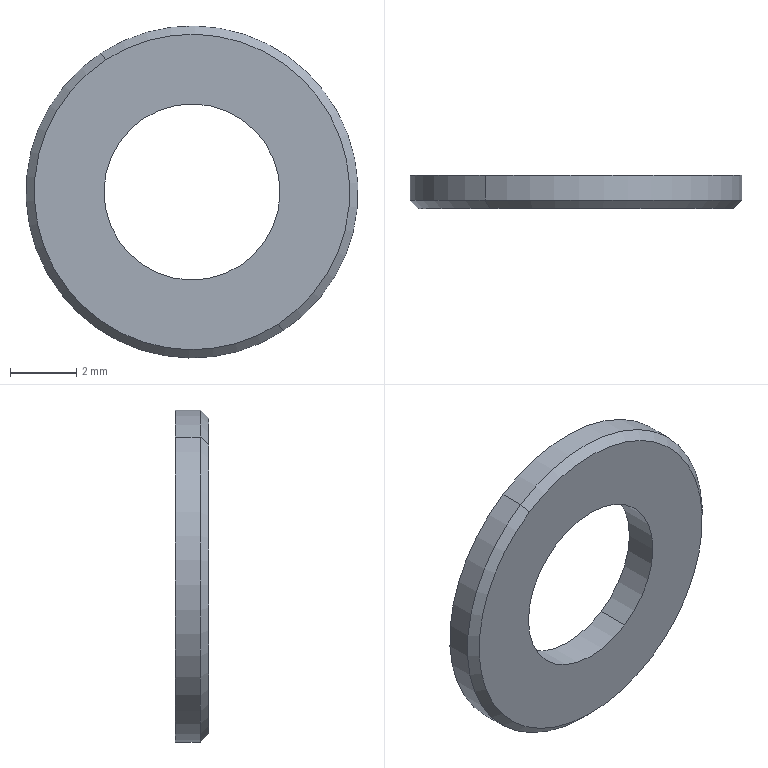Component | SolidWorks | GB_T97.2-1985FlatWasherChamferedTypeA5_1-4 | 1 solid | 8 faces | box 10 x 1 x 10 mm | volume 56 mm3 | cylinder 4 | cone 2 | plane 2 | commonest cylinder face diameters 10 x2 5.3 x2 | material AISI 321 Annealed Stainless Steel (SS)
build123d program:
from build123d import *


with BuildPart() as part:
    # Sketch1 → Base-Revolve (revolve)
    with BuildSketch(Plane.XY, mode=Mode.PRIVATE) as base_revolve_sk:
        Polygon((-4.75, 9.645), (-5, 9.395), (-5, 8.645), (-2.65, 8.645), (-2.65, 9.645), align=None)
    revolve(base_revolve_sk.sketch.rotate(Axis((0, 0, 0), (0, 1, 0)), 270), axis=Axis((0, 0, 0), (0, 1, 0)))


solid = part.part

# Placed as in the assembly
solid = solid.moved(Location((-239.428, 163.441, 253.382), (180, 0, 0)))